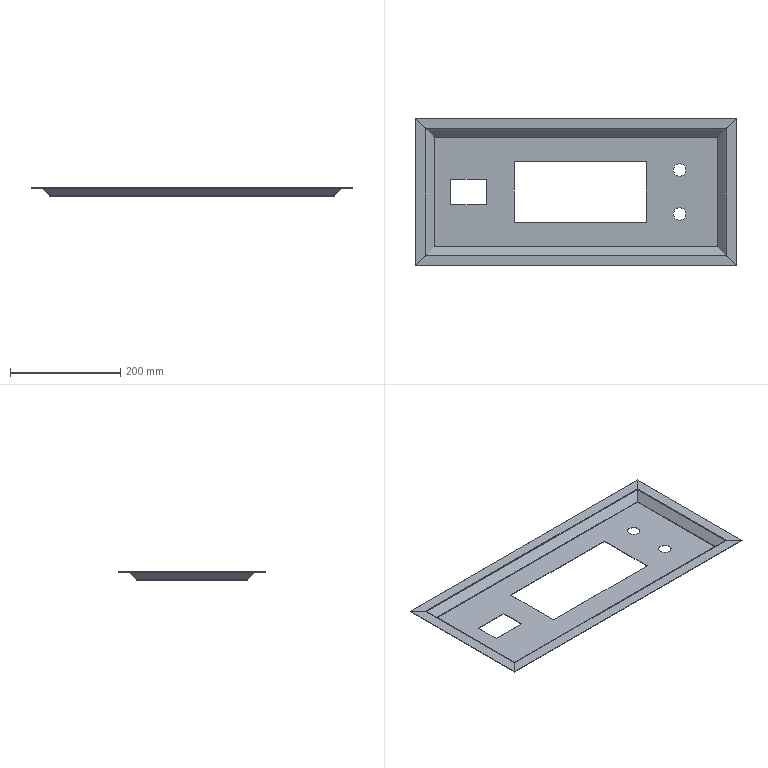Component | SolidWorks | CCQ-1.1-10Panel-1 | 1 solid | 82 faces | volume 134728 mm3 | plane 46 | cylinder 20 | spline 16 | commonest cylinder face diameters 3.473 x8 1.473 x8 22.5 x4 | material 304